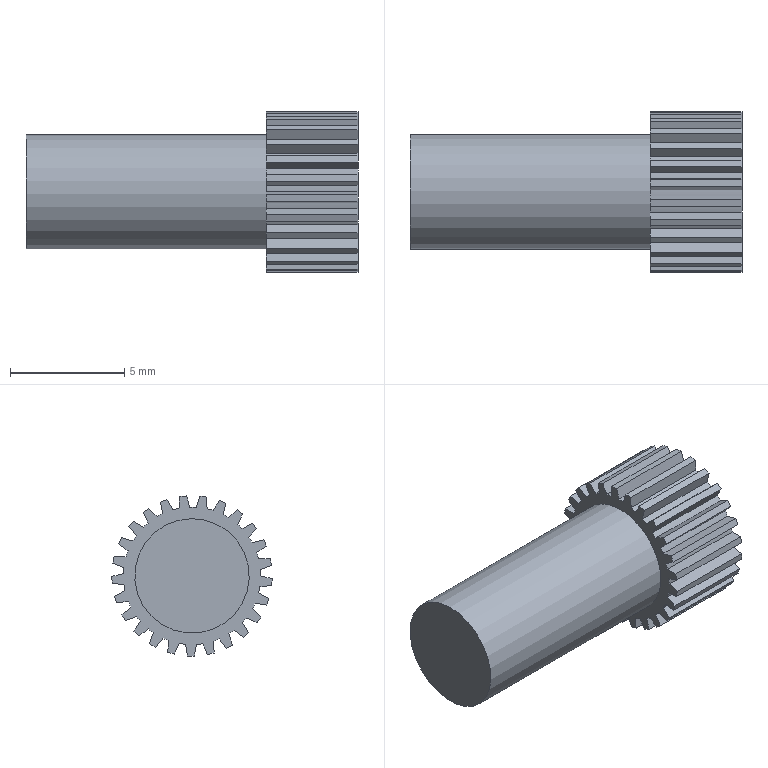Component | NX | LOCKING_KNOB | 1 solid | 104 faces | volume 339 mm3 | plane 78 | cylinder 26 | commonest cylinder face diameters 6 x25 5 x1